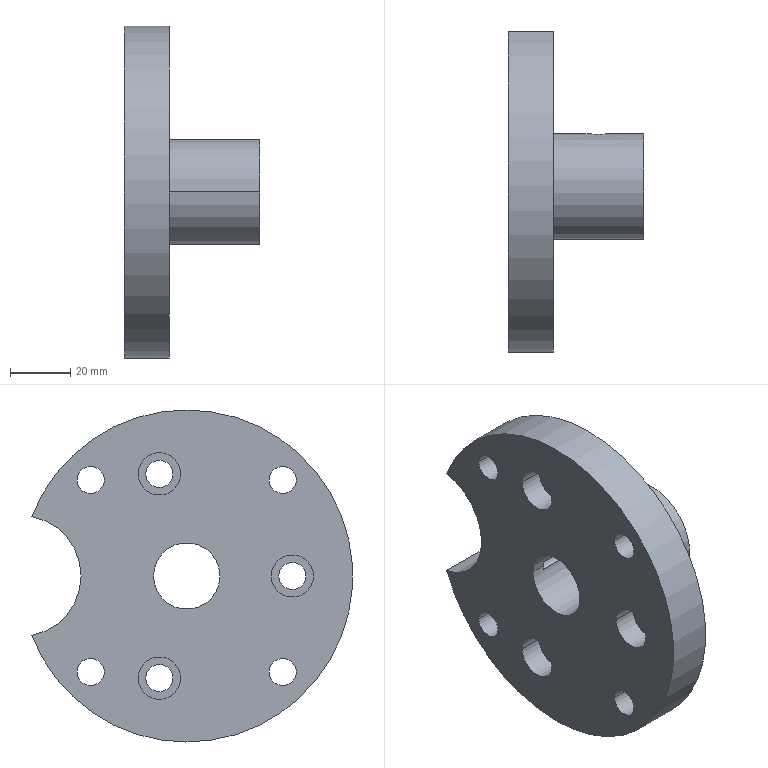Component | SolidWorks | 6IndexingPlate-1 | 1 solid | 41 faces | volume 136526 mm3 | cylinder 33 | plane 8 | commonest cylinder face diameters 9 x14 14 x6 3 x4 5 x2 40 x2 22 x2 35 x2 110 x1